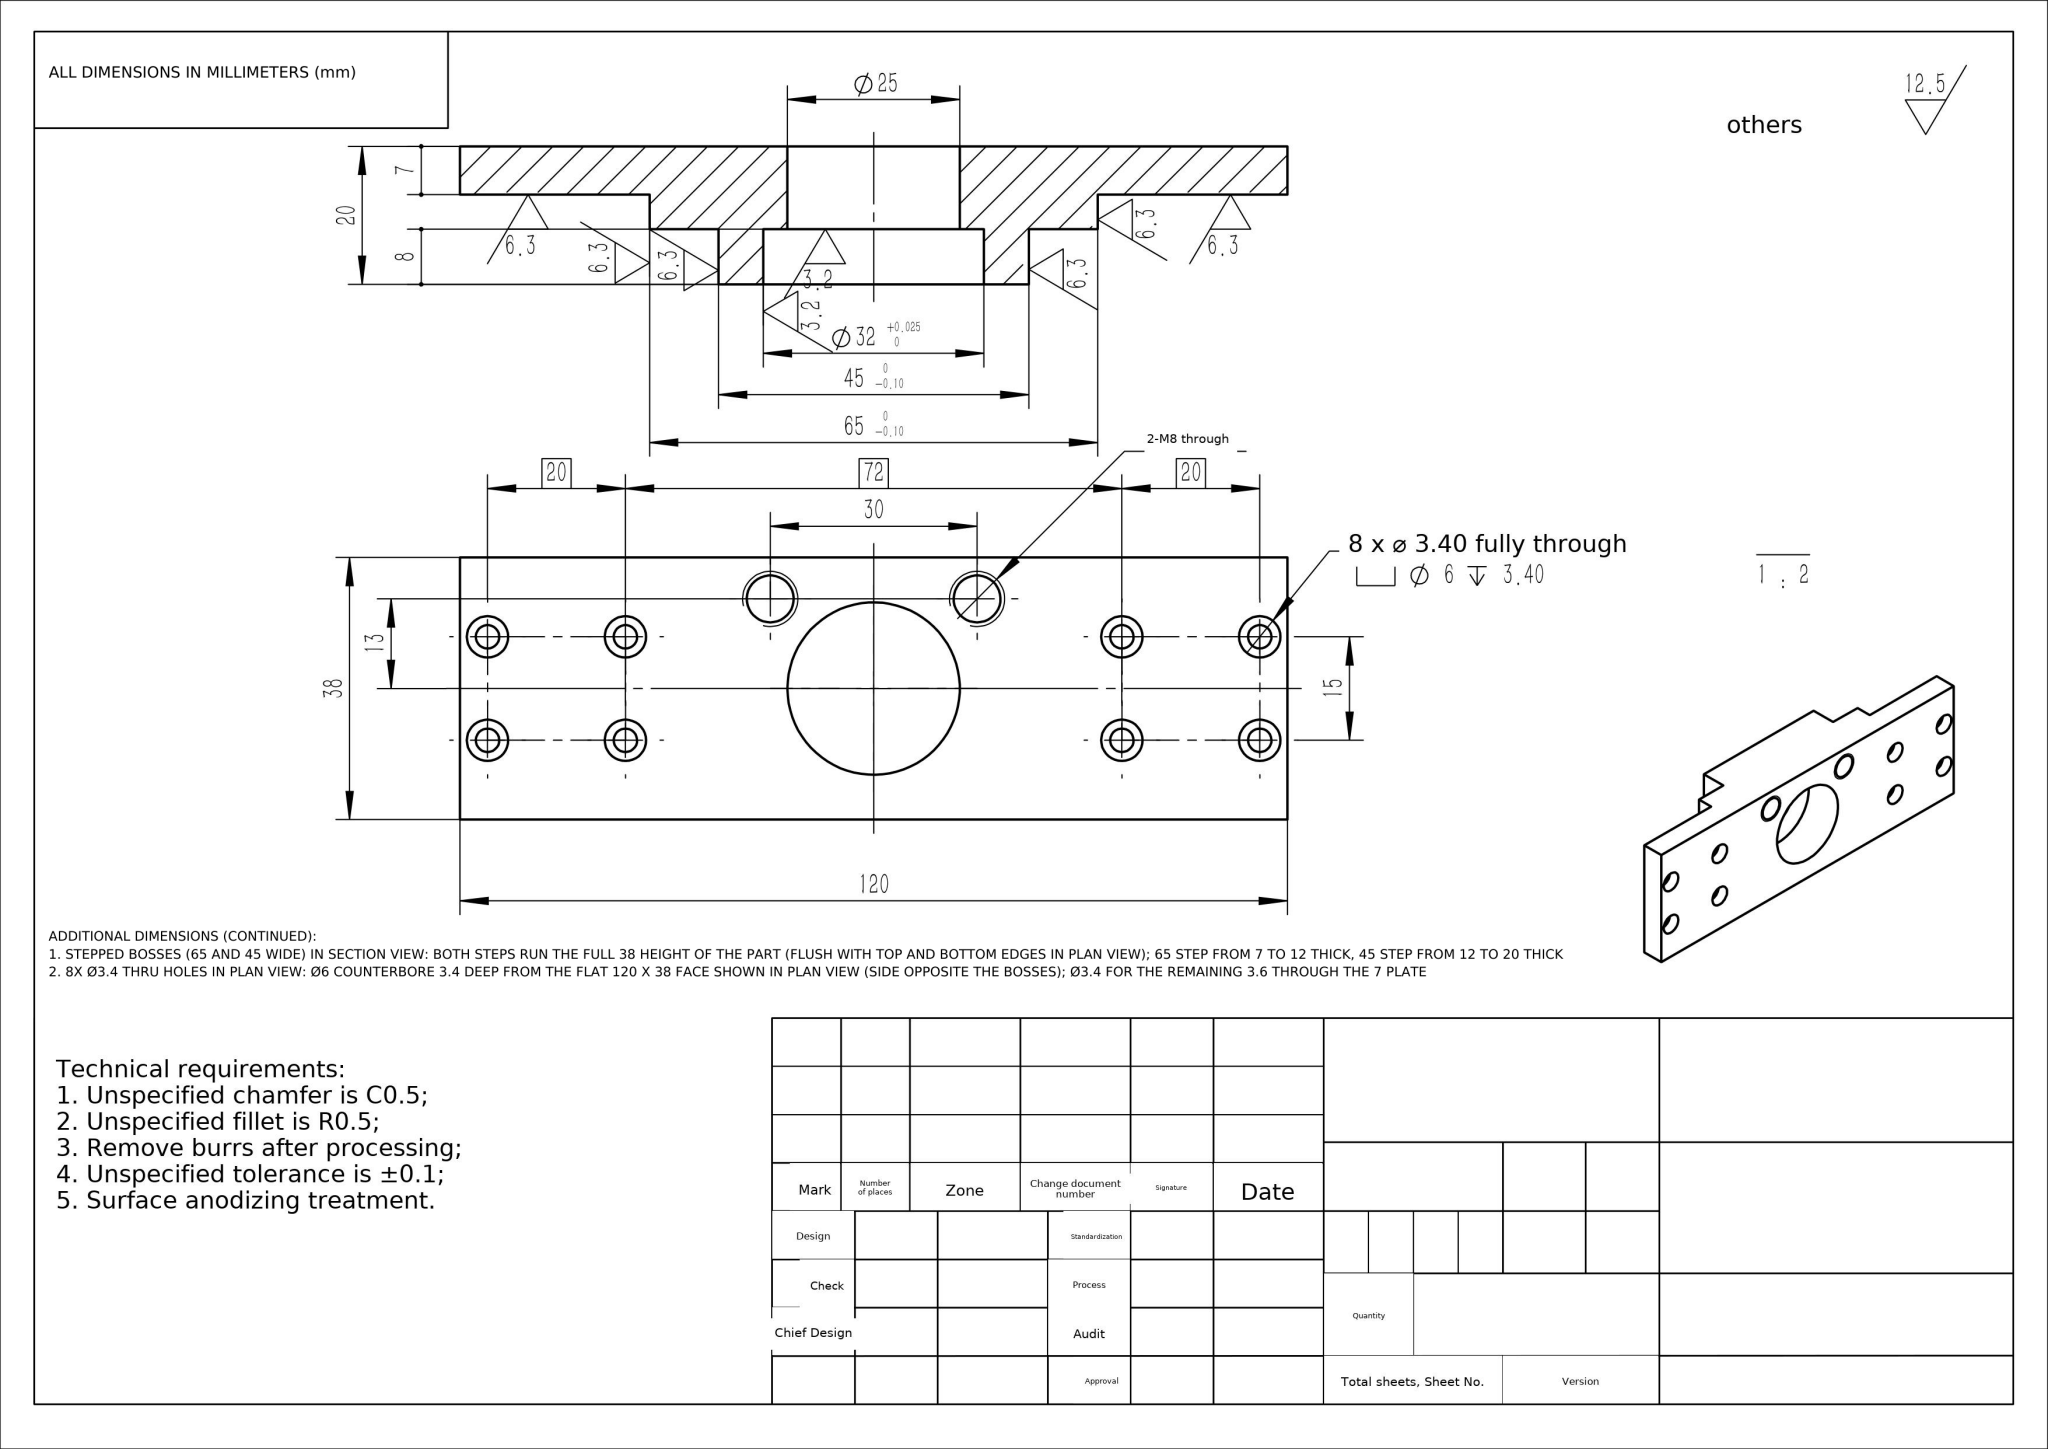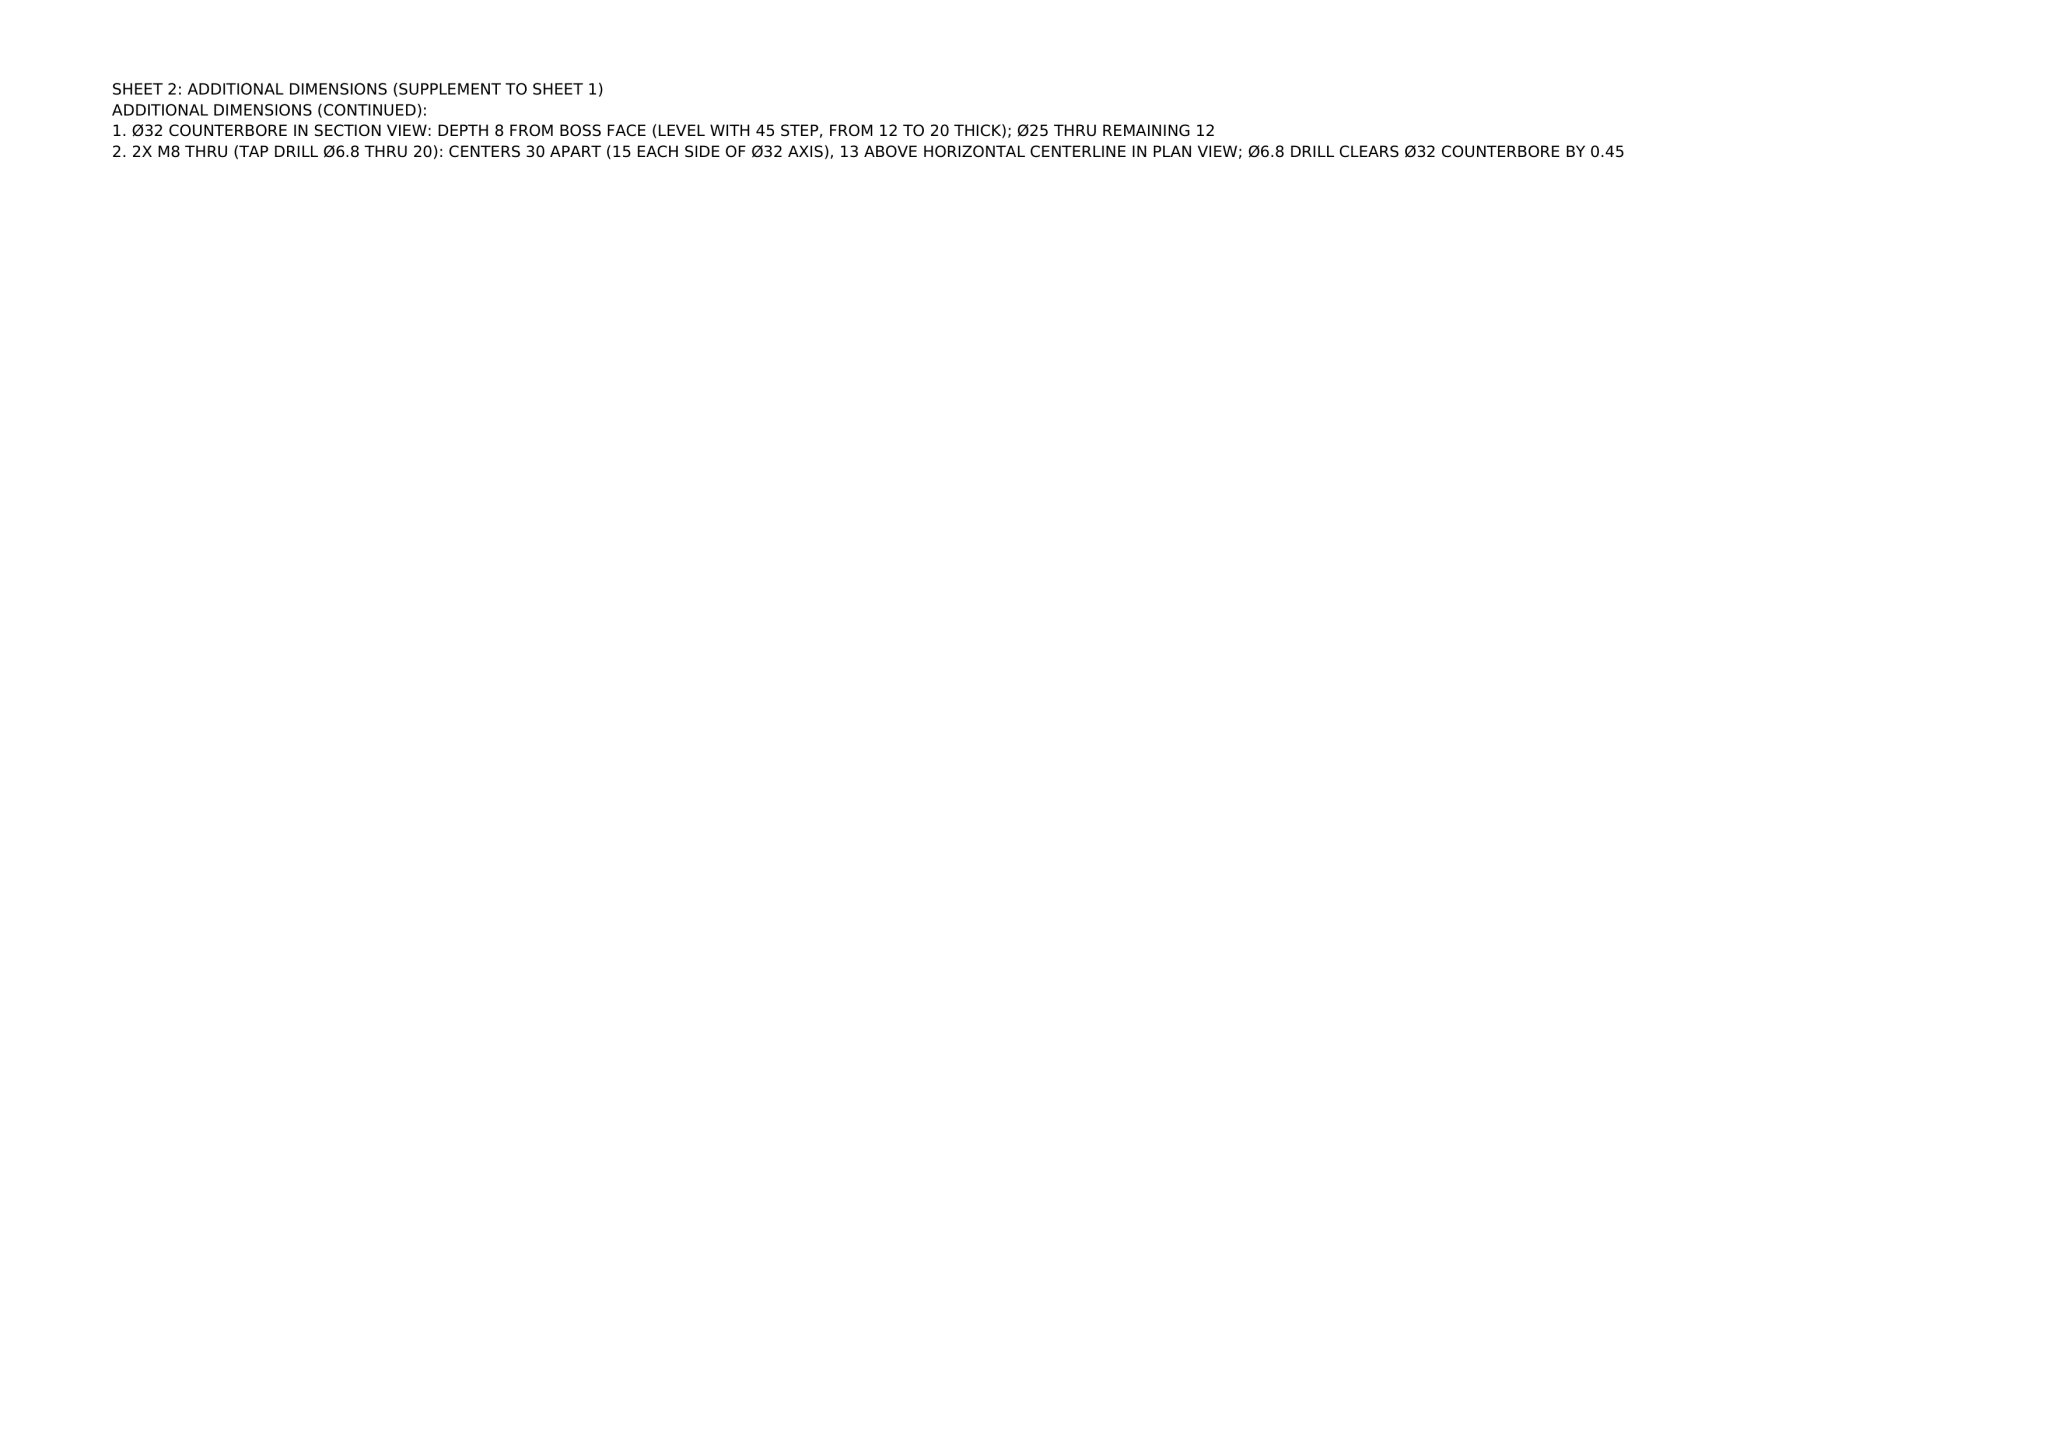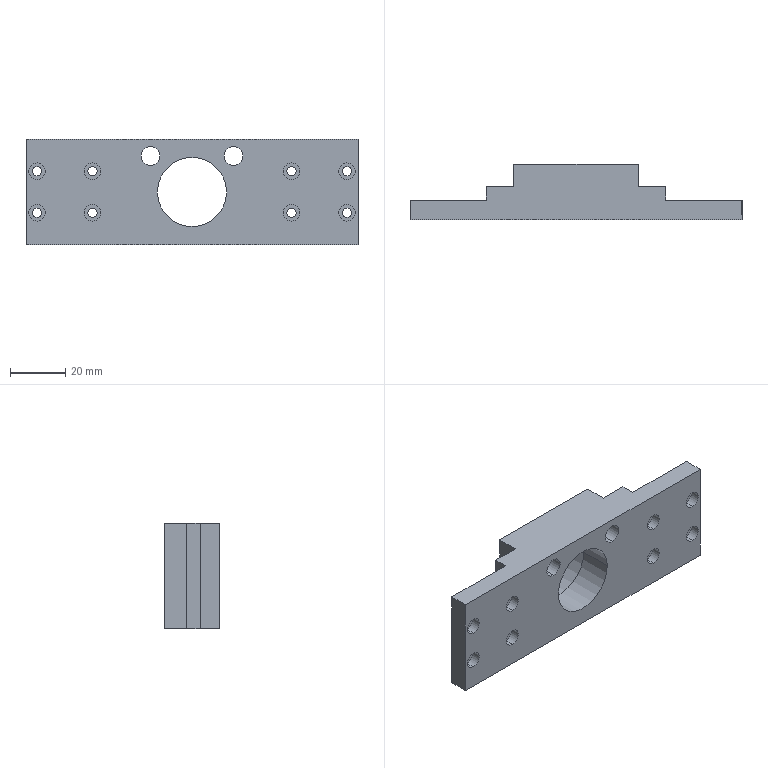Part | NX | mm | 1 solid | 63 faces | box 120 x 20 x 38 mm | volume 43142 mm3 | cylinder 40 | plane 23 | commonest cylinder face diameters 6 x16 3.4 x16 6.8 x4 25 x2 32 x2